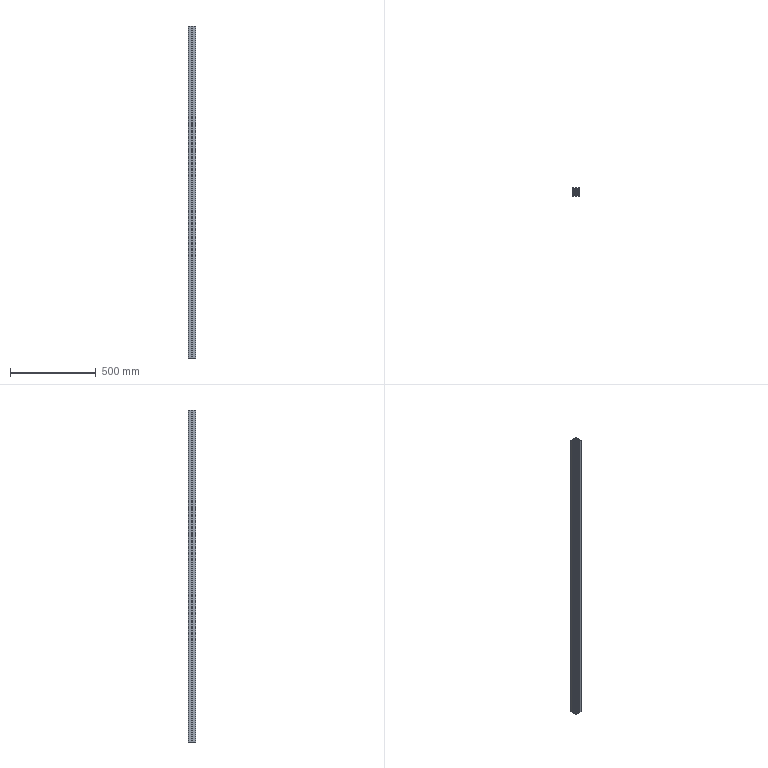Component | SolidWorks | HFS8_4545_01-B-1 | 1 solid | 131 faces | box 45 x 45 x 1932 mm | volume 1549851 mm3 | plane 82 | cylinder 49 | commonest cylinder face diameters 2 x18 3 x12 1 x10 12.5 x5 6 x4 | material 6061-T4 (SS)
build123d program:
from build123d import *

# Parameters (mm, degrees)
BOSS_EXTRUDE1_DEPTH = 1932


with BuildPart() as part:
    # Sketch1 → Boss-Extrude1 (new body)
    with BuildSketch(Plane.XY):
        with BuildLine():
            Line((-19.5, -22.5), (-5, -22.5))
            Line((-5, -22.5), (-5, -16.5))
            Line((-5, -16.5), (-10, -16.5))
            Line((-10, -16.5), (-10, -13))
            Line((-10, -13), (-6.5, -9.5))
            Line((-6.5, -9.5), (-1.212, -9.5))
            Line((-1.212, -9.5), (0, -8.8))
            Line((0, -8.8), (1.212, -9.5))
            Line((1.212, -9.5), (6.5, -9.5))
            Line((6.5, -9.5), (10, -13))
            Line((10, -13), (10, -16.5))
            Line((10, -16.5), (5, -16.5))
            Line((5, -16.5), (5, -22.5))
            Line((5, -22.5), (19.5, -22.5))
            ThreePointArc((19.5, -22.5), (21.621, -21.621), (22.5, -19.5))
            Line((22.5, -19.5), (22.5, -5))
            Line((22.5, -5), (16.5, -5))
            Line((16.5, -5), (16.5, -10))
            Line((16.5, -10), (13, -10))
            Line((13, -10), (9.5, -6.5))
            Line((9.5, -6.5), (9.5, -1.212))
            Line((9.5, -1.212), (8.8, 0))
            Line((8.8, 0), (9.5, 1.212))
            Line((9.5, 1.212), (9.5, 6.5))
            Line((9.5, 6.5), (13, 10))
            Line((13, 10), (16.5, 10))
            Line((16.5, 10), (16.5, 5))
            Line((16.5, 5), (22.5, 5))
            Line((22.5, 5), (22.5, 19.5))
            ThreePointArc((22.5, 19.5), (21.621, 21.621), (19.5, 22.5))
            Line((19.5, 22.5), (5, 22.5))
            Line((5, 22.5), (5, 16.5))
            Line((5, 16.5), (10, 16.5))
            Line((10, 16.5), (10, 13))
            Line((10, 13), (6.5, 9.5))
            Line((6.5, 9.5), (1.212, 9.5))
            Line((1.212, 9.5), (0, 8.8))
            Line((0, 8.8), (-1.212, 9.5))
            Line((-1.212, 9.5), (-6.5, 9.5))
            Line((-6.5, 9.5), (-10, 13))
            Line((-10, 13), (-10, 16.5))
            Line((-10, 16.5), (-5, 16.5))
            Line((-5, 16.5), (-5, 22.5))
            Line((-5, 22.5), (-19.5, 22.5))
            ThreePointArc((-19.5, 22.5), (-21.621, 21.621), (-22.5, 19.5))
            Line((-22.5, 19.5), (-22.5, 5))
            Line((-22.5, 5), (-16.5, 5))
            Line((-16.5, 5), (-16.5, 10))
            Line((-16.5, 10), (-13, 10))
            Line((-13, 10), (-9.5, 6.5))
            Line((-9.5, 6.5), (-9.5, 1.212))
            Line((-9.5, 1.212), (-8.8, 0))
            Line((-8.8, 0), (-9.5, -1.212))
            Line((-9.5, -1.212), (-9.5, -6.5))
            Line((-9.5, -6.5), (-13, -10))
            Line((-13, -10), (-16.5, -10))
            Line((-16.5, -10), (-16.5, -5))
            Line((-16.5, -5), (-22.5, -5))
            Line((-22.5, -5), (-22.5, -19.5))
            ThreePointArc((-22.5, -19.5), (-21.621, -21.621), (-19.5, -22.5))
        make_face()
        with BuildLine():
            Line((12, 18.5), (12, 13))
            ThreePointArc((12, 13), (12.293, 12.293), (13, 12))
            Line((13, 12), (18.5, 12))
            ThreePointArc((18.5, 12), (19.5, 11), (20.5, 12))
            Line((20.5, 12), (20.5, 19.5))
            ThreePointArc((20.5, 19.5), (20.207, 20.207), (19.5, 20.5))
            Line((19.5, 20.5), (12, 20.5))
            ThreePointArc((12, 20.5), (11, 19.5), (12, 18.5))
        make_face(mode=Mode.SUBTRACT)
        with BuildLine():
            Line((12, -20.5), (19.5, -20.5))
            ThreePointArc((19.5, -20.5), (20.207, -20.207), (20.5, -19.5))
            Line((20.5, -19.5), (20.5, -12))
            ThreePointArc((20.5, -12), (19.5, -11), (18.5, -12))
            Line((18.5, -12), (13, -12))
            ThreePointArc((13, -12), (12.293, -12.293), (12, -13))
            Line((12, -13), (12, -18.5))
            ThreePointArc((12, -18.5), (11, -19.5), (12, -20.5))
        make_face(mode=Mode.SUBTRACT)
        with BuildLine():
            Line((-4.725, -6.139), (-3.947, -5.361))
            ThreePointArc((-3.947, -5.361), (-3.649, -5.217), (-3.327, -5.291))
            ThreePointArc((-3.327, -5.291), (0, -6.25), (3.327, -5.291))
            ThreePointArc((3.327, -5.291), (3.649, -5.217), (3.947, -5.361))
            Line((3.947, -5.361), (4.725, -6.139))
            ThreePointArc((4.725, -6.139), (7.283, -7.283), (6.139, -4.725))
            Line((6.139, -4.725), (5.361, -3.947))
            ThreePointArc((5.361, -3.947), (5.217, -3.649), (5.291, -3.327))
            ThreePointArc((5.291, -3.327), (6.25, 0), (5.291, 3.327))
            ThreePointArc((5.291, 3.327), (5.217, 3.649), (5.361, 3.947))
            Line((5.361, 3.947), (6.139, 4.725))
            ThreePointArc((6.139, 4.725), (7.283, 7.283), (4.725, 6.139))
            Line((4.725, 6.139), (3.947, 5.361))
            ThreePointArc((3.947, 5.361), (3.649, 5.217), (3.327, 5.291))
            ThreePointArc((3.327, 5.291), (0, 6.25), (-3.327, 5.291))
            ThreePointArc((-3.327, 5.291), (-3.649, 5.217), (-3.947, 5.361))
            Line((-3.947, 5.361), (-4.725, 6.139))
            ThreePointArc((-4.725, 6.139), (-7.283, 7.283), (-6.139, 4.725))
            Line((-6.139, 4.725), (-5.361, 3.947))
            ThreePointArc((-5.361, 3.947), (-5.217, 3.649), (-5.291, 3.327))
            ThreePointArc((-5.291, 3.327), (-6.25, 0), (-5.291, -3.327))
            ThreePointArc((-5.291, -3.327), (-5.217, -3.649), (-5.361, -3.947))
            Line((-5.361, -3.947), (-6.139, -4.725))
            ThreePointArc((-6.139, -4.725), (-7.283, -7.283), (-4.725, -6.139))
        make_face(mode=Mode.SUBTRACT)
        with BuildLine():
            Line((-19.5, -20.5), (-12, -20.5))
            ThreePointArc((-12, -20.5), (-11, -19.5), (-12, -18.5))
            Line((-12, -18.5), (-12, -13))
            ThreePointArc((-12, -13), (-12.293, -12.293), (-13, -12))
            Line((-13, -12), (-18.5, -12))
            ThreePointArc((-18.5, -12), (-19.5, -11), (-20.5, -12))
            Line((-20.5, -12), (-20.5, -19.5))
            ThreePointArc((-20.5, -19.5), (-20.207, -20.207), (-19.5, -20.5))
        make_face(mode=Mode.SUBTRACT)
        with BuildLine():
            Line((-18.5, 12), (-13, 12))
            ThreePointArc((-13, 12), (-12.293, 12.293), (-12, 13))
            Line((-12, 13), (-12, 18.5))
            ThreePointArc((-12, 18.5), (-11, 19.5), (-12, 20.5))
            Line((-12, 20.5), (-19.5, 20.5))
            ThreePointArc((-19.5, 20.5), (-20.207, 20.207), (-20.5, 19.5))
            Line((-20.5, 19.5), (-20.5, 12))
            ThreePointArc((-20.5, 12), (-19.5, 11), (-18.5, 12))
        make_face(mode=Mode.SUBTRACT)
    extrude(amount=-BOSS_EXTRUDE1_DEPTH)


solid = part.part

# Placed as in the assembly
solid = solid.moved(Location((-65.506, 8.087, -470.928), (0, 0, 0)))